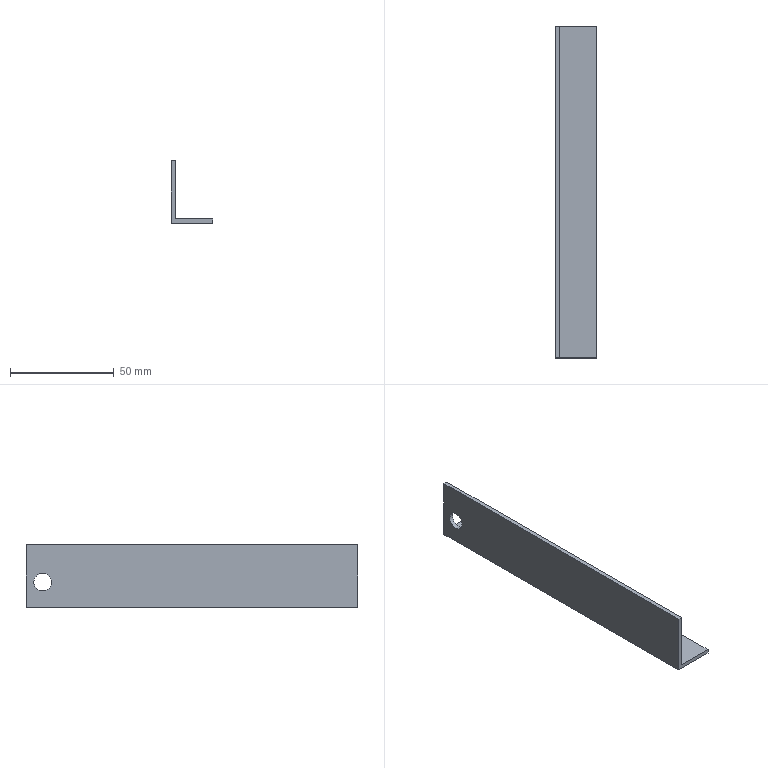Component | SolidWorks | KSD171005A-01-01-31-1 | 1 solid | 10 faces | box 20 x 160 x 30 mm | volume 15247 mm3 | plane 8 | cylinder 2 | commonest cylinder face diameters 8.5 x2
build123d program:
from build123d import *

# Parameters (mm, degrees)
EXTRUDE_THIN1_DEPTH            = 80
F_8_5_8_5_DIAMETER_HOLE2_D     = 8.5
F_8_5_8_5_DIAMETER_HOLE2_DEPTH = 11
F_8_5_8_5_DIAMETER_HOLE2_TIP   = 2.554


with BuildPart() as part:
    # Sketch1 → Extrude-Thin1 (new, symmetric)
    with BuildSketch(Plane.XY):
        Polygon((30, 0), (0, 0), (0, 20), (2, 20), (2, 2), (30, 2), align=None)
    extrude(amount=EXTRUDE_THIN1_DEPTH, both=True)

    # 8.5 _8.5_ Diameter Hole2
    with Locations(Plane(origin=(0, 0, 0), x_dir=(-1, 0, 0), z_dir=(0, -1, 0))):
        with Locations((-12, -72)):
            Hole(F_8_5_8_5_DIAMETER_HOLE2_D / 2, depth=F_8_5_8_5_DIAMETER_HOLE2_DEPTH)
            with Locations((0, 0, -(F_8_5_8_5_DIAMETER_HOLE2_DEPTH + F_8_5_8_5_DIAMETER_HOLE2_TIP / 2))):  # 118° drill point
                Cone(0, F_8_5_8_5_DIAMETER_HOLE2_D / 2, F_8_5_8_5_DIAMETER_HOLE2_TIP, mode=Mode.SUBTRACT)


solid = part.part

# Placed as in the assembly
solid = solid.moved(Location((-21.611, -73.27, 395), (-90, 0, -90)))
STEP:
#1=CARTESIAN_POINT('',(-0.7721,0.1173,16.024));
#2=VERTEX_POINT('',#1);
#3=CARTESIAN_POINT('',(-0.7721,-0.2173,16.024));
#4=VERTEX_POINT('',#3);
#5=CARTESIAN_POINT('',(-0.7721,-0.05001,16.024));
#6=DIRECTION('',(-1.,-0.,0.));
#7=DIRECTION('',(0.,0.,1.));
#8=AXIS2_PLACEMENT_3D('',#5,#6,#7);
#9=CIRCLE('',#8,0.1673);
#10=EDGE_CURVE('',#2,#4,#9,.T.);
#11=ORIENTED_EDGE('',*,*,#10,.F.);
#12=CARTESIAN_POINT('',(-0.8508,0.1173,16.024));
#13=VERTEX_POINT('',#12);
#14=CARTESIAN_POINT('',(-0.8508,0.1173,16.024));
#15=DIRECTION('',(-1.,-0.,0.));
#16=VECTOR('',#15,39.37);
#17=LINE('',#14,#16);
#18=EDGE_CURVE('',#2,#13,#17,.T.);
#19=ORIENTED_EDGE('',*,*,#18,.T.);
#20=CARTESIAN_POINT('',(-0.8508,-0.2173,16.024));
#21=VERTEX_POINT('',#20);
#22=CARTESIAN_POINT('',(-0.8508,-0.05001,16.024));
#23=DIRECTION('',(-1.,-0.,0.));
#24=DIRECTION('',(0.,-1.,0.));
#25=AXIS2_PLACEMENT_3D('',#22,#23,#24);
#26=CIRCLE('',#25,0.1673);
#27=EDGE_CURVE('',#13,#21,#26,.T.);
#28=ORIENTED_EDGE('',*,*,#27,.T.);
#29=CARTESIAN_POINT('',(-0.8508,-0.2173,16.024));
#30=DIRECTION('',(-1.,-0.,0.));
#31=VECTOR('',#30,39.37);
#32=LINE('',#29,#31);
#33=EDGE_CURVE('',#4,#21,#32,.T.);
#34=ORIENTED_EDGE('',*,*,#33,.F.);
#35=EDGE_LOOP('',(#11,#19,#28,#34));
#36=FACE_OUTER_BOUND('',#35,.T.);
#37=CARTESIAN_POINT('',(-0.8508,-0.05001,16.024));
#38=DIRECTION('',(-1.,-0.,0.));
#39=DIRECTION('',(0.,-1.,0.));
#40=AXIS2_PLACEMENT_3D('',#37,#38,#39);
#41=CYLINDRICAL_SURFACE('',#40,0.1673);
#42=ADVANCED_FACE('',(#36),#41,.F.);
#43=CARTESIAN_POINT('',(-0.7721,-6.034,15.63));
#44=VERTEX_POINT('',#43);
#45=CARTESIAN_POINT('',(-0.06344,-6.034,15.63));
#46=VERTEX_POINT('',#45);
#47=CARTESIAN_POINT('',(-0.8508,-6.034,15.63));
#48=DIRECTION('',(1.,0.,-0.));
#49=VECTOR('',#48,39.37);
#50=LINE('',#47,#49);
#51=EDGE_CURVE('',#44,#46,#50,.T.);
#52=ORIENTED_EDGE('',*,*,#51,.T.);
#53=CARTESIAN_POINT('',(-0.06344,0.265,15.63));
#54=VERTEX_POINT('',#53);
#55=CARTESIAN_POINT('',(-0.06344,0.265,15.63));
#56=DIRECTION('',(0.,-1.,0.));
#57=VECTOR('',#56,39.37);
#58=LINE('',#55,#57);
#59=EDGE_CURVE('',#54,#46,#58,.T.);
#60=ORIENTED_EDGE('',*,*,#59,.F.);
#61=CARTESIAN_POINT('',(-0.7721,0.265,15.63));
#62=VERTEX_POINT('',#61);
#63=CARTESIAN_POINT('',(-0.8508,0.265,15.63));
#64=DIRECTION('',(1.,0.,-0.));
#65=VECTOR('',#64,39.37);
#66=LINE('',#63,#65);
#67=EDGE_CURVE('',#62,#54,#66,.T.);
#68=ORIENTED_EDGE('',*,*,#67,.F.);
#69=CARTESIAN_POINT('',(-0.7721,0.265,15.63));
#70=DIRECTION('',(0.,-1.,0.));
#71=VECTOR('',#70,39.37);
#72=LINE('',#69,#71);
#73=EDGE_CURVE('',#62,#44,#72,.T.);
#74=ORIENTED_EDGE('',*,*,#73,.T.);
#75=EDGE_LOOP('',(#52,#60,#68,#74));
#76=FACE_OUTER_BOUND('',#75,.T.);
#77=CARTESIAN_POINT('',(-0.8508,0.265,15.63));
#78=DIRECTION('',(0.,-0.,-1.));
#79=DIRECTION('',(-0.,1.,-0.));
#80=AXIS2_PLACEMENT_3D('',#77,#78,#79);
#81=PLANE('',#80);
#82=ADVANCED_FACE('',(#76),#81,.F.);
#83=CARTESIAN_POINT('',(-0.06344,-6.034,15.551));
#84=VERTEX_POINT('',#83);
#85=CARTESIAN_POINT('',(-0.06344,-6.034,15.551));
#86=DIRECTION('',(-0.,0.,1.));
#87=VECTOR('',#86,39.37);
#88=LINE('',#85,#87);
#89=EDGE_CURVE('',#84,#46,#88,.T.);
#90=ORIENTED_EDGE('',*,*,#89,.F.);
#91=CARTESIAN_POINT('',(-0.06344,0.265,15.551));
#92=VERTEX_POINT('',#91);
#93=CARTESIAN_POINT('',(-0.06344,0.265,15.551));
#94=DIRECTION('',(0.,-1.,0.));
#95=VECTOR('',#94,39.37);
#96=LINE('',#93,#95);
#97=EDGE_CURVE('',#92,#84,#96,.T.);
#98=ORIENTED_EDGE('',*,*,#97,.F.);
#99=CARTESIAN_POINT('',(-0.06344,0.265,15.551));
#100=DIRECTION('',(-0.,0.,1.));
#101=VECTOR('',#100,39.37);
#102=LINE('',#99,#101);
#103=EDGE_CURVE('',#92,#54,#102,.T.);
#104=ORIENTED_EDGE('',*,*,#103,.T.);
#105=ORIENTED_EDGE('',*,*,#59,.T.);
#106=EDGE_LOOP('',(#90,#98,#104,#105));
#107=FACE_OUTER_BOUND('',#106,.T.);
#108=CARTESIAN_POINT('',(-0.06344,0.265,15.551));
#109=DIRECTION('',(1.,0.,-0.));
#110=DIRECTION('',(-0.,1.,-0.));
#111=AXIS2_PLACEMENT_3D('',#108,#109,#110);
#112=PLANE('',#111);
#113=ADVANCED_FACE('',(#107),#112,.T.);
#114=CARTESIAN_POINT('',(-0.8508,-6.034,15.551));
#115=VERTEX_POINT('',#114);
#116=CARTESIAN_POINT('',(-0.8508,-6.034,15.551));
#117=DIRECTION('',(1.,0.,-0.));
#118=VECTOR('',#117,39.37);
#119=LINE('',#116,#118);
#120=EDGE_CURVE('',#115,#84,#119,.T.);
#121=ORIENTED_EDGE('',*,*,#120,.F.);
#122=CARTESIAN_POINT('',(-0.8508,0.265,15.551));
#123=VERTEX_POINT('',#122);
#124=CARTESIAN_POINT('',(-0.8508,0.265,15.551));
#125=DIRECTION('',(0.,-1.,0.));
#126=VECTOR('',#125,39.37);
#127=LINE('',#124,#126);
#128=EDGE_CURVE('',#123,#115,#127,.T.);
#129=ORIENTED_EDGE('',*,*,#128,.F.);
#130=CARTESIAN_POINT('',(-0.8508,0.265,15.551));
#131=DIRECTION('',(1.,0.,-0.));
#132=VECTOR('',#131,39.37);
#133=LINE('',#130,#132);
#134=EDGE_CURVE('',#123,#92,#133,.T.);
#135=ORIENTED_EDGE('',*,*,#134,.T.);
#136=ORIENTED_EDGE('',*,*,#97,.T.);
#137=EDGE_LOOP('',(#121,#129,#135,#136));
#138=FACE_OUTER_BOUND('',#137,.T.);
#139=CARTESIAN_POINT('',(-0.8508,0.265,15.551));
#140=DIRECTION('',(0.,-0.,-1.));
#141=DIRECTION('',(-0.,1.,-0.));
#142=AXIS2_PLACEMENT_3D('',#139,#140,#141);
#143=PLANE('',#142);
#144=ADVANCED_FACE('',(#138),#143,.T.);
#145=CARTESIAN_POINT('',(-0.8508,-0.05001,16.024));
#146=DIRECTION('',(-1.,-0.,0.));
#147=DIRECTION('',(0.,-1.,0.));
#148=AXIS2_PLACEMENT_3D('',#145,#146,#147);
#149=CIRCLE('',#148,0.1673);
#150=EDGE_CURVE('',#21,#13,#149,.T.);
#151=ORIENTED_EDGE('',*,*,#150,.F.);
#152=ORIENTED_EDGE('',*,*,#27,.F.);
#153=EDGE_LOOP('',(#151,#152));
#154=FACE_BOUND('',#153,.T.);
#155=CARTESIAN_POINT('',(-0.8508,-6.034,16.732));
#156=VERTEX_POINT('',#155);
#157=CARTESIAN_POINT('',(-0.8508,-6.034,16.732));
#158=DIRECTION('',(-0.,-0.,-1.));
#159=VECTOR('',#158,39.37);
#160=LINE('',#157,#159);
#161=EDGE_CURVE('',#156,#115,#160,.T.);
#162=ORIENTED_EDGE('',*,*,#161,.F.);
#163=CARTESIAN_POINT('',(-0.8508,0.265,16.732));
#164=VERTEX_POINT('',#163);
#165=CARTESIAN_POINT('',(-0.8508,0.265,16.732));
#166=DIRECTION('',(0.,-1.,0.));
#167=VECTOR('',#166,39.37);
#168=LINE('',#165,#167);
#169=EDGE_CURVE('',#164,#156,#168,.T.);
#170=ORIENTED_EDGE('',*,*,#169,.F.);
#171=CARTESIAN_POINT('',(-0.8508,0.265,16.732));
#172=DIRECTION('',(-0.,-0.,-1.));
#173=VECTOR('',#172,39.37);
#174=LINE('',#171,#173);
#175=EDGE_CURVE('',#164,#123,#174,.T.);
#176=ORIENTED_EDGE('',*,*,#175,.T.);
#177=ORIENTED_EDGE('',*,*,#128,.T.);
#178=EDGE_LOOP('',(#162,#170,#176,#177));
#179=FACE_OUTER_BOUND('',#178,.T.);
#180=CARTESIAN_POINT('',(-0.8508,0.265,16.732));
#181=DIRECTION('',(-1.,-0.,0.));
#182=DIRECTION('',(0.,0.,1.));
#183=AXIS2_PLACEMENT_3D('',#180,#181,#182);
#184=PLANE('',#183);
#185=ADVANCED_FACE('',(#154,#179),#184,.T.);
#186=CARTESIAN_POINT('',(-0.7721,-6.034,16.732));
#187=VERTEX_POINT('',#186);
#188=CARTESIAN_POINT('',(-0.7721,-6.034,16.732));
#189=DIRECTION('',(-1.,-0.,0.));
#190=VECTOR('',#189,39.37);
#191=LINE('',#188,#190);
#192=EDGE_CURVE('',#187,#156,#191,.T.);
#193=ORIENTED_EDGE('',*,*,#192,.F.);
#194=CARTESIAN_POINT('',(-0.7721,0.265,16.732));
#195=VERTEX_POINT('',#194);
#196=CARTESIAN_POINT('',(-0.7721,0.265,16.732));
#197=DIRECTION('',(0.,-1.,0.));
#198=VECTOR('',#197,39.37);
#199=LINE('',#196,#198);
#200=EDGE_CURVE('',#195,#187,#199,.T.);
#201=ORIENTED_EDGE('',*,*,#200,.F.);
#202=CARTESIAN_POINT('',(-0.7721,0.265,16.732));
#203=DIRECTION('',(-1.,-0.,0.));
#204=VECTOR('',#203,39.37);
#205=LINE('',#202,#204);
#206=EDGE_CURVE('',#195,#164,#205,.T.);
#207=ORIENTED_EDGE('',*,*,#206,.T.);
#208=ORIENTED_EDGE('',*,*,#169,.T.);
#209=EDGE_LOOP('',(#193,#201,#207,#208));
#210=FACE_OUTER_BOUND('',#209,.T.);
#211=CARTESIAN_POINT('',(-0.7721,0.265,16.732));
#212=DIRECTION('',(-0.,0.,1.));
#213=DIRECTION('',(0.,-1.,0.));
#214=AXIS2_PLACEMENT_3D('',#211,#212,#213);
#215=PLANE('',#214);
#216=ADVANCED_FACE('',(#210),#215,.T.);
#217=CARTESIAN_POINT('',(-0.7721,-0.05001,16.024));
#218=DIRECTION('',(-1.,-0.,0.));
#219=DIRECTION('',(0.,0.,1.));
#220=AXIS2_PLACEMENT_3D('',#217,#218,#219);
#221=CIRCLE('',#220,0.1673);
#222=EDGE_CURVE('',#4,#2,#221,.T.);
#223=ORIENTED_EDGE('',*,*,#222,.T.);
#224=ORIENTED_EDGE('',*,*,#10,.T.);
#225=EDGE_LOOP('',(#223,#224));
#226=FACE_BOUND('',#225,.T.);
#227=CARTESIAN_POINT('',(-0.7721,-6.034,16.732));
#228=DIRECTION('',(-0.,-0.,-1.));
#229=VECTOR('',#228,39.37);
#230=LINE('',#227,#229);
#231=EDGE_CURVE('',#187,#44,#230,.T.);
#232=ORIENTED_EDGE('',*,*,#231,.T.);
#233=ORIENTED_EDGE('',*,*,#73,.F.);
#234=CARTESIAN_POINT('',(-0.7721,0.265,16.732));
#235=DIRECTION('',(-0.,-0.,-1.));
#236=VECTOR('',#235,39.37);
#237=LINE('',#234,#236);
#238=EDGE_CURVE('',#195,#62,#237,.T.);
#239=ORIENTED_EDGE('',*,*,#238,.F.);
#240=ORIENTED_EDGE('',*,*,#200,.T.);
#241=EDGE_LOOP('',(#232,#233,#239,#240));
#242=FACE_OUTER_BOUND('',#241,.T.);
#243=CARTESIAN_POINT('',(-0.7721,0.265,16.732));
#244=DIRECTION('',(-1.,-0.,0.));
#245=DIRECTION('',(0.,0.,1.));
#246=AXIS2_PLACEMENT_3D('',#243,#244,#245);
#247=PLANE('',#246);
#248=ADVANCED_FACE('',(#226,#242),#247,.F.);
#249=ORIENTED_EDGE('',*,*,#67,.T.);
#250=ORIENTED_EDGE('',*,*,#103,.F.);
#251=ORIENTED_EDGE('',*,*,#134,.F.);
#252=ORIENTED_EDGE('',*,*,#175,.F.);
#253=ORIENTED_EDGE('',*,*,#206,.F.);
#254=ORIENTED_EDGE('',*,*,#238,.T.);
#255=EDGE_LOOP('',(#249,#250,#251,#252,#253,#254));
#256=FACE_OUTER_BOUND('',#255,.T.);
#257=CARTESIAN_POINT('',(-0.8508,0.265,15.551));
#258=DIRECTION('',(0.,-1.,0.));
#259=DIRECTION('',(0.,-0.,-1.));
#260=AXIS2_PLACEMENT_3D('',#257,#258,#259);
#261=PLANE('',#260);
#262=ADVANCED_FACE('',(#256),#261,.F.);
#263=ORIENTED_EDGE('',*,*,#51,.F.);
#264=ORIENTED_EDGE('',*,*,#231,.F.);
#265=ORIENTED_EDGE('',*,*,#192,.T.);
#266=ORIENTED_EDGE('',*,*,#161,.T.);
#267=ORIENTED_EDGE('',*,*,#120,.T.);
#268=ORIENTED_EDGE('',*,*,#89,.T.);
#269=EDGE_LOOP('',(#263,#264,#265,#266,#267,#268));
#270=FACE_OUTER_BOUND('',#269,.T.);
#271=CARTESIAN_POINT('',(-0.8508,-6.034,15.551));
#272=DIRECTION('',(0.,-1.,0.));
#273=DIRECTION('',(0.,-0.,-1.));
#274=AXIS2_PLACEMENT_3D('',#271,#272,#273);
#275=PLANE('',#274);
#276=ADVANCED_FACE('',(#270),#275,.T.);
#277=ORIENTED_EDGE('',*,*,#18,.F.);
#278=ORIENTED_EDGE('',*,*,#222,.F.);
#279=ORIENTED_EDGE('',*,*,#33,.T.);
#280=ORIENTED_EDGE('',*,*,#150,.T.);
#281=EDGE_LOOP('',(#277,#278,#279,#280));
#282=FACE_OUTER_BOUND('',#281,.T.);
#283=CARTESIAN_POINT('',(-0.8508,-0.05001,16.024));
#284=DIRECTION('',(-1.,-0.,0.));
#285=DIRECTION('',(0.,-1.,0.));
#286=AXIS2_PLACEMENT_3D('',#283,#284,#285);
#287=CYLINDRICAL_SURFACE('',#286,0.1673);
#288=ADVANCED_FACE('',(#282),#287,.F.);
#289=CLOSED_SHELL('',(#42,#82,#113,#144,#185,#216,#248,#262,#276,#288));
#290=MANIFOLD_SOLID_BREP('',#289);
#291=CARTESIAN_POINT('',(0.,0.,0.));
#292=DIRECTION('',(0.,0.,1.));
#293=DIRECTION('',(1.,0.,0.));
#294=AXIS2_PLACEMENT_3D('',#291,#292,#293);
#295=(LENGTH_UNIT()NAMED_UNIT(*)SI_UNIT($,.METRE.));
#296=LENGTH_MEASURE_WITH_UNIT(LENGTH_MEASURE(0.0254),#295);
#297=DIMENSIONAL_EXPONENTS(1.,0.,0.,0.,0.,0.,0.);
#298=(CONVERSION_BASED_UNIT('',#296)LENGTH_UNIT()NAMED_UNIT(#297));
#299=UNCERTAINTY_MEASURE_WITH_UNIT(LENGTH_MEASURE(0.00001),#298,'','');
#300=(NAMED_UNIT(*)PLANE_ANGLE_UNIT()SI_UNIT($,.RADIAN.));
#301=(NAMED_UNIT(*)SI_UNIT($,.STERADIAN.)SOLID_ANGLE_UNIT());
#302=(GEOMETRIC_REPRESENTATION_CONTEXT(3)GLOBAL_UNCERTAINTY_ASSIGNED_CONTEXT((#299))GLOBAL_UNIT_ASSIGNED_CONTEXT((#298,#300,#301))REPRESENTATION_CONTEXT('',''));
#303=ADVANCED_BREP_SHAPE_REPRESENTATION('',(#290,#294),#302);
#304=COLOUR_RGB('',0.7922,0.8196,0.9333);
#305=FILL_AREA_STYLE_COLOUR('',#304);
#306=FILL_AREA_STYLE('',(#305));
#307=SURFACE_STYLE_FILL_AREA(#306);
#308=SURFACE_SIDE_STYLE('',(#307));
#309=SURFACE_STYLE_USAGE(.BOTH.,#308);
#310=PRESENTATION_STYLE_ASSIGNMENT((#309));
#311=STYLED_ITEM('',(#310),#290);
#312=(LENGTH_UNIT()NAMED_UNIT(*)SI_UNIT($,.METRE.));
#313=LENGTH_MEASURE_WITH_UNIT(LENGTH_MEASURE(0.0254),#312);
#314=DIMENSIONAL_EXPONENTS(1.,0.,0.,0.,0.,0.,0.);
#315=(CONVERSION_BASED_UNIT('',#313)LENGTH_UNIT()NAMED_UNIT(#314));
#316=UNCERTAINTY_MEASURE_WITH_UNIT(LENGTH_MEASURE(0.00001),#315,'','');
#317=(NAMED_UNIT(*)PLANE_ANGLE_UNIT()SI_UNIT($,.RADIAN.));
#318=(NAMED_UNIT(*)SI_UNIT($,.STERADIAN.)SOLID_ANGLE_UNIT());
#319=(GEOMETRIC_REPRESENTATION_CONTEXT(3)GLOBAL_UNCERTAINTY_ASSIGNED_CONTEXT((#316))GLOBAL_UNIT_ASSIGNED_CONTEXT((#315,#317,#318))REPRESENTATION_CONTEXT('',''));
#320=MECHANICAL_DESIGN_GEOMETRIC_PRESENTATION_REPRESENTATION('',(#311),#319);
#321=PRESENTATION_LAYER_ASSIGNMENT('','',(#311));